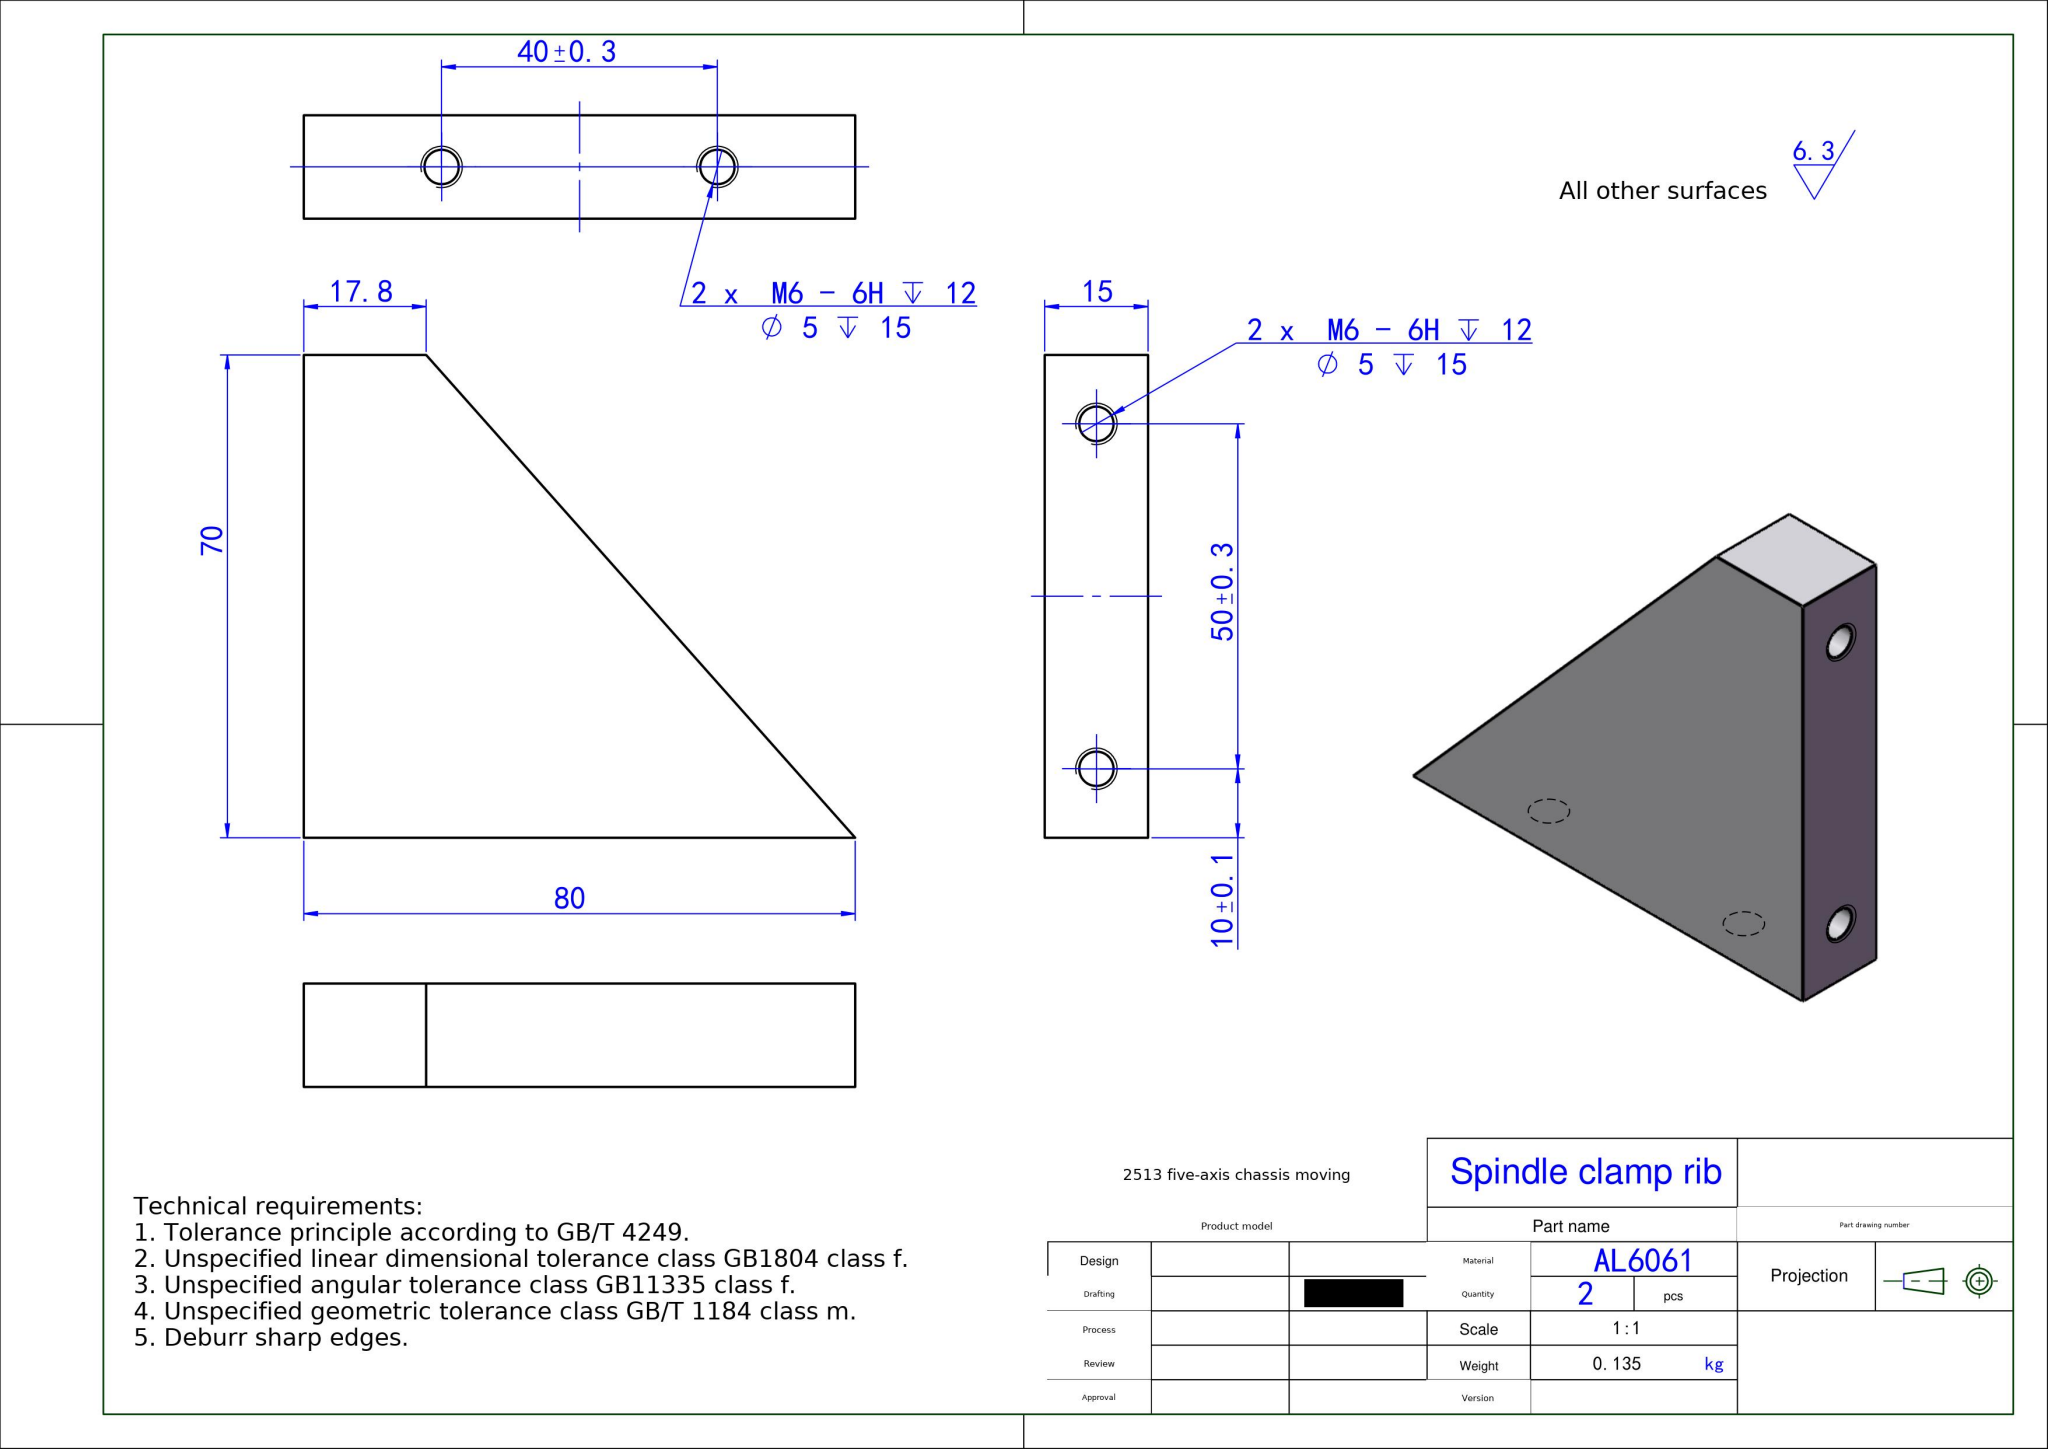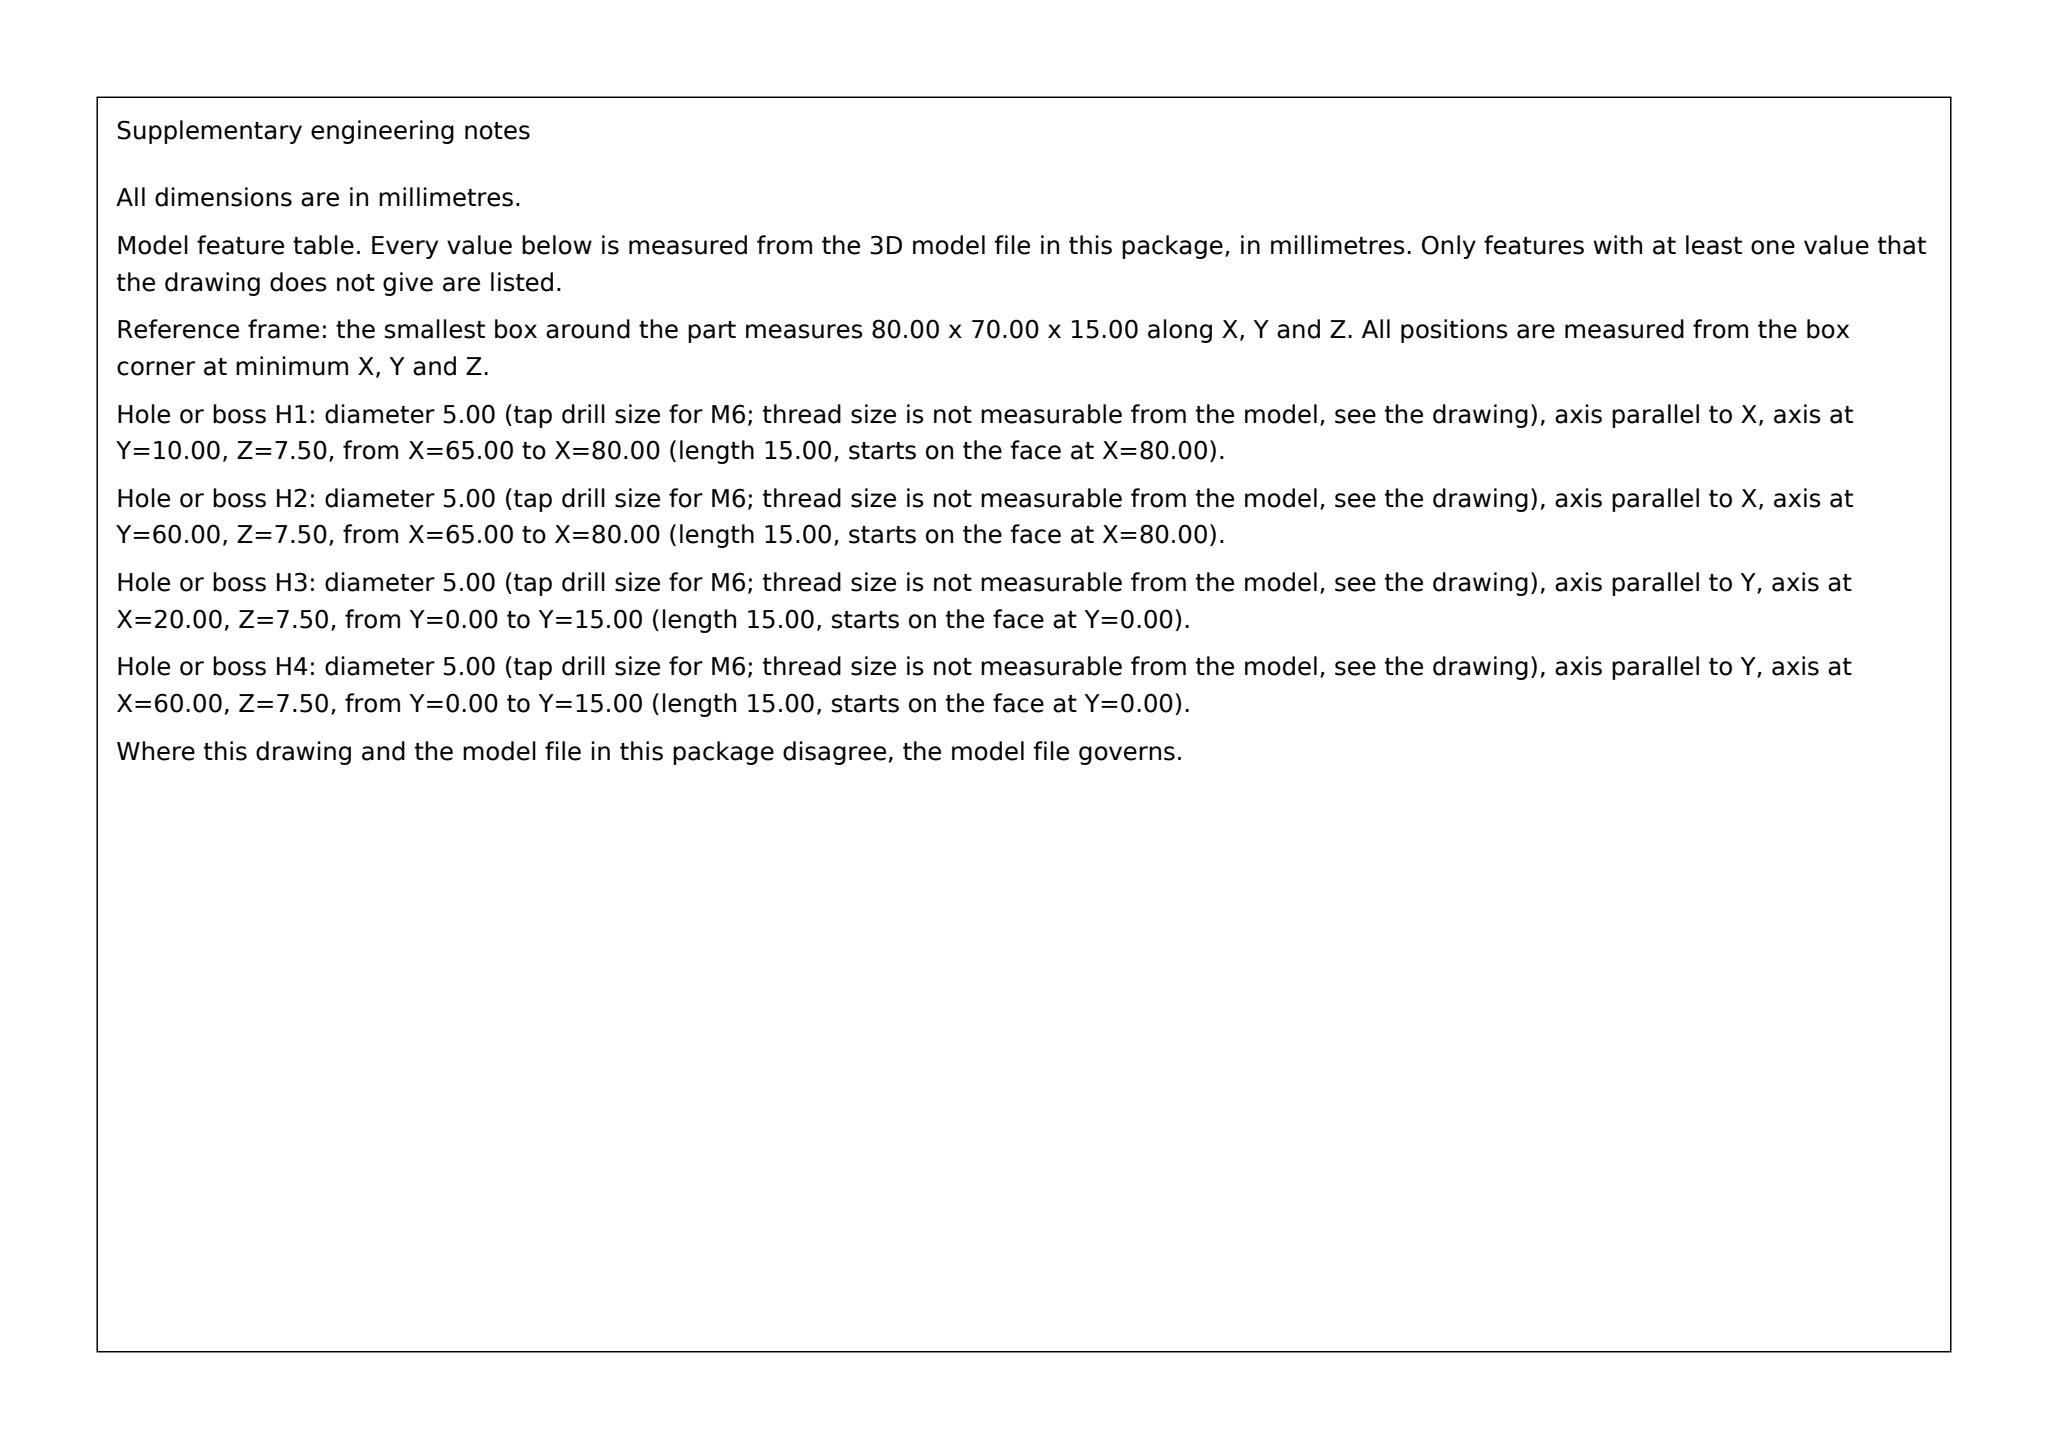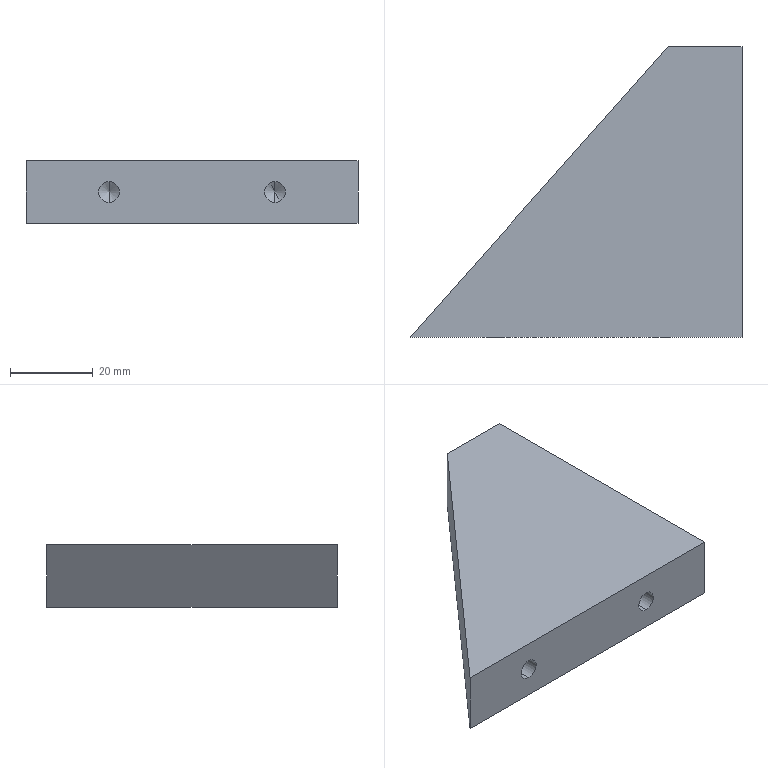Part | SolidWorks | mm | material AL6061 | 1 solid | 22 faces | box 80 x 70 x 15 mm | volume 50116 mm3 | cylinder 8 | cone 8 | plane 6 | commonest cylinder face diameters 5 x8
build123d program:
from build123d import *

# Parameters (mm, degrees)
BOSS_EXTRUDE1_DEPTH   = 15
CUT_EXTRUDE1_DEPTH    = 15
M6_TAPPED_HOLE1_D     = 5
M6_TAPPED_HOLE1_DEPTH = 15
M6_TAPPED_HOLE1_TIP   = 1.502
M6_TAPPED_HOLE2_D     = 5
M6_TAPPED_HOLE2_DEPTH = 15
M6_TAPPED_HOLE2_TIP   = 1.502


with BuildPart() as part:
    # Sketch1 → Boss-Extrude1 (new body)
    with BuildSketch(Plane.XY):
        Polygon((-23, -46), (-103, -136), (-23, -136), align=None)
    extrude(amount=-BOSS_EXTRUDE1_DEPTH)

    # Sketch2 → Cut-Extrude1 (cut)
    with BuildSketch(Plane.XY):
        Polygon((-40.778, -66), (-23, -66), (-23, -46), align=None)
    extrude(amount=-CUT_EXTRUDE1_DEPTH, mode=Mode.SUBTRACT)

    # M6 Tapped Hole1
    with Locations(Plane(origin=(-23, 0, 0), x_dir=(0, 0, -1), z_dir=(1, 0, 0))):
        with Locations((7.5, -76), (7.5, -126)):
            Hole(M6_TAPPED_HOLE1_D / 2, depth=M6_TAPPED_HOLE1_DEPTH)
            with Locations((0, 0, -(M6_TAPPED_HOLE1_DEPTH + M6_TAPPED_HOLE1_TIP / 2))):  # 118° drill point
                Cone(0, M6_TAPPED_HOLE1_D / 2, M6_TAPPED_HOLE1_TIP, mode=Mode.SUBTRACT)

    # M6 Tapped Hole2
    with Locations(Plane(origin=(0, -136, 0), x_dir=(-1, 0, 0), z_dir=(0, -1, 0))):
        with Locations((43, 7.5), (83, 7.5)):
            Hole(M6_TAPPED_HOLE2_D / 2, depth=M6_TAPPED_HOLE2_DEPTH)
            with Locations((0, 0, -(M6_TAPPED_HOLE2_DEPTH + M6_TAPPED_HOLE2_TIP / 2))):  # 118° drill point
                Cone(0, M6_TAPPED_HOLE2_D / 2, M6_TAPPED_HOLE2_TIP, mode=Mode.SUBTRACT)


solid = part.part
STEP:
#1=CARTESIAN_POINT('',(-43.,-121.,-5.));
#2=VERTEX_POINT('',#1);
#3=CARTESIAN_POINT('',(-43.,-121.,-10.));
#4=VERTEX_POINT('',#3);
#5=CARTESIAN_POINT('',(-43.,-121.,-7.5));
#6=DIRECTION('',(0.,-1.,0.));
#7=DIRECTION('',(0.,0.,-1.));
#8=AXIS2_PLACEMENT_3D('',#5,#6,#7);
#9=CIRCLE('',#8,2.5);
#10=EDGE_CURVE('',#2,#4,#9,.T.);
#11=ORIENTED_EDGE('',*,*,#10,.F.);
#12=CARTESIAN_POINT('',(-43.,-136.,-5.));
#13=VERTEX_POINT('',#12);
#14=CARTESIAN_POINT('',(-43.,-136.,-5.));
#15=DIRECTION('',(0.,-1.,0.));
#16=VECTOR('',#15,1000.);
#17=LINE('',#14,#16);
#18=EDGE_CURVE('',#2,#13,#17,.T.);
#19=ORIENTED_EDGE('',*,*,#18,.T.);
#20=CARTESIAN_POINT('',(-43.,-136.,-10.));
#21=VERTEX_POINT('',#20);
#22=CARTESIAN_POINT('',(-43.,-136.,-7.5));
#23=DIRECTION('',(0.,-1.,0.));
#24=DIRECTION('',(0.,0.,-1.));
#25=AXIS2_PLACEMENT_3D('',#22,#23,#24);
#26=CIRCLE('',#25,2.5);
#27=EDGE_CURVE('',#13,#21,#26,.T.);
#28=ORIENTED_EDGE('',*,*,#27,.T.);
#29=CARTESIAN_POINT('',(-43.,-136.,-10.));
#30=DIRECTION('',(0.,-1.,0.));
#31=VECTOR('',#30,1000.);
#32=LINE('',#29,#31);
#33=EDGE_CURVE('',#4,#21,#32,.T.);
#34=ORIENTED_EDGE('',*,*,#33,.F.);
#35=EDGE_LOOP('',(#11,#19,#28,#34));
#36=FACE_OUTER_BOUND('',#35,.T.);
#37=CARTESIAN_POINT('',(-43.,-136.,-7.5));
#38=DIRECTION('',(0.,-1.,0.));
#39=DIRECTION('',(0.,0.,-1.));
#40=AXIS2_PLACEMENT_3D('',#37,#38,#39);
#41=CYLINDRICAL_SURFACE('',#40,2.5);
#42=ADVANCED_FACE('',(#36),#41,.F.);
#43=CARTESIAN_POINT('',(-43.,-119.498,-7.5));
#44=VERTEX_POINT('',#43);
#45=CARTESIAN_POINT('',(-43.,-121.,-10.));
#46=DIRECTION('',(0.,-0.515,-0.8572));
#47=VECTOR('',#46,1000.);
#48=LINE('',#45,#47);
#49=EDGE_CURVE('',#44,#4,#48,.T.);
#50=ORIENTED_EDGE('',*,*,#49,.F.);
#51=CARTESIAN_POINT('',(-43.,-121.,-5.));
#52=DIRECTION('',(0.,-0.515,0.8572));
#53=VECTOR('',#52,1000.);
#54=LINE('',#51,#53);
#55=EDGE_CURVE('',#44,#2,#54,.T.);
#56=ORIENTED_EDGE('',*,*,#55,.T.);
#57=ORIENTED_EDGE('',*,*,#10,.T.);
#58=EDGE_LOOP('',(#50,#56,#57));
#59=FACE_OUTER_BOUND('',#58,.T.);
#60=CARTESIAN_POINT('',(-43.,-121.,-7.5));
#61=DIRECTION('',(0.,-1.,0.));
#62=DIRECTION('',(0.,0.,-1.));
#63=AXIS2_PLACEMENT_3D('',#60,#61,#62);
#64=CONICAL_SURFACE('',#63,2.5,1.03);
#65=ADVANCED_FACE('',(#59),#64,.F.);
#66=CARTESIAN_POINT('',(-83.,-121.,-5.));
#67=VERTEX_POINT('',#66);
#68=CARTESIAN_POINT('',(-83.,-121.,-10.));
#69=VERTEX_POINT('',#68);
#70=CARTESIAN_POINT('',(-83.,-121.,-7.5));
#71=DIRECTION('',(0.,-1.,0.));
#72=DIRECTION('',(0.,0.,-1.));
#73=AXIS2_PLACEMENT_3D('',#70,#71,#72);
#74=CIRCLE('',#73,2.5);
#75=EDGE_CURVE('',#67,#69,#74,.T.);
#76=ORIENTED_EDGE('',*,*,#75,.F.);
#77=CARTESIAN_POINT('',(-83.,-136.,-5.));
#78=VERTEX_POINT('',#77);
#79=CARTESIAN_POINT('',(-83.,-136.,-5.));
#80=DIRECTION('',(0.,-1.,0.));
#81=VECTOR('',#80,1000.);
#82=LINE('',#79,#81);
#83=EDGE_CURVE('',#67,#78,#82,.T.);
#84=ORIENTED_EDGE('',*,*,#83,.T.);
#85=CARTESIAN_POINT('',(-83.,-136.,-10.));
#86=VERTEX_POINT('',#85);
#87=CARTESIAN_POINT('',(-83.,-136.,-7.5));
#88=DIRECTION('',(0.,-1.,0.));
#89=DIRECTION('',(0.,0.,-1.));
#90=AXIS2_PLACEMENT_3D('',#87,#88,#89);
#91=CIRCLE('',#90,2.5);
#92=EDGE_CURVE('',#78,#86,#91,.T.);
#93=ORIENTED_EDGE('',*,*,#92,.T.);
#94=CARTESIAN_POINT('',(-83.,-136.,-10.));
#95=DIRECTION('',(0.,-1.,0.));
#96=VECTOR('',#95,1000.);
#97=LINE('',#94,#96);
#98=EDGE_CURVE('',#69,#86,#97,.T.);
#99=ORIENTED_EDGE('',*,*,#98,.F.);
#100=EDGE_LOOP('',(#76,#84,#93,#99));
#101=FACE_OUTER_BOUND('',#100,.T.);
#102=CARTESIAN_POINT('',(-83.,-136.,-7.5));
#103=DIRECTION('',(0.,-1.,0.));
#104=DIRECTION('',(0.,0.,-1.));
#105=AXIS2_PLACEMENT_3D('',#102,#103,#104);
#106=CYLINDRICAL_SURFACE('',#105,2.5);
#107=ADVANCED_FACE('',(#101),#106,.F.);
#108=CARTESIAN_POINT('',(-83.,-119.498,-7.5));
#109=VERTEX_POINT('',#108);
#110=CARTESIAN_POINT('',(-83.,-121.,-10.));
#111=DIRECTION('',(0.,-0.515,-0.8572));
#112=VECTOR('',#111,1000.);
#113=LINE('',#110,#112);
#114=EDGE_CURVE('',#109,#69,#113,.T.);
#115=ORIENTED_EDGE('',*,*,#114,.F.);
#116=CARTESIAN_POINT('',(-83.,-121.,-5.));
#117=DIRECTION('',(0.,-0.515,0.8572));
#118=VECTOR('',#117,1000.);
#119=LINE('',#116,#118);
#120=EDGE_CURVE('',#109,#67,#119,.T.);
#121=ORIENTED_EDGE('',*,*,#120,.T.);
#122=ORIENTED_EDGE('',*,*,#75,.T.);
#123=EDGE_LOOP('',(#115,#121,#122));
#124=FACE_OUTER_BOUND('',#123,.T.);
#125=CARTESIAN_POINT('',(-83.,-121.,-7.5));
#126=DIRECTION('',(0.,-1.,0.));
#127=DIRECTION('',(0.,0.,-1.));
#128=AXIS2_PLACEMENT_3D('',#125,#126,#127);
#129=CONICAL_SURFACE('',#128,2.5,1.03);
#130=ADVANCED_FACE('',(#124),#129,.F.);
#131=CARTESIAN_POINT('',(-38.,-76.,-5.));
#132=VERTEX_POINT('',#131);
#133=CARTESIAN_POINT('',(-38.,-76.,-10.));
#134=VERTEX_POINT('',#133);
#135=CARTESIAN_POINT('',(-38.,-76.,-7.5));
#136=DIRECTION('',(1.,0.,0.));
#137=DIRECTION('',(0.,0.,-1.));
#138=AXIS2_PLACEMENT_3D('',#135,#136,#137);
#139=CIRCLE('',#138,2.5);
#140=EDGE_CURVE('',#132,#134,#139,.T.);
#141=ORIENTED_EDGE('',*,*,#140,.F.);
#142=CARTESIAN_POINT('',(-23.,-76.,-5.));
#143=VERTEX_POINT('',#142);
#144=CARTESIAN_POINT('',(-23.,-76.,-5.));
#145=DIRECTION('',(1.,0.,0.));
#146=VECTOR('',#145,1000.);
#147=LINE('',#144,#146);
#148=EDGE_CURVE('',#132,#143,#147,.T.);
#149=ORIENTED_EDGE('',*,*,#148,.T.);
#150=CARTESIAN_POINT('',(-23.,-76.,-10.));
#151=VERTEX_POINT('',#150);
#152=CARTESIAN_POINT('',(-23.,-76.,-7.5));
#153=DIRECTION('',(1.,0.,0.));
#154=DIRECTION('',(0.,0.,-1.));
#155=AXIS2_PLACEMENT_3D('',#152,#153,#154);
#156=CIRCLE('',#155,2.5);
#157=EDGE_CURVE('',#143,#151,#156,.T.);
#158=ORIENTED_EDGE('',*,*,#157,.T.);
#159=CARTESIAN_POINT('',(-23.,-76.,-10.));
#160=DIRECTION('',(1.,0.,0.));
#161=VECTOR('',#160,1000.);
#162=LINE('',#159,#161);
#163=EDGE_CURVE('',#134,#151,#162,.T.);
#164=ORIENTED_EDGE('',*,*,#163,.F.);
#165=EDGE_LOOP('',(#141,#149,#158,#164));
#166=FACE_OUTER_BOUND('',#165,.T.);
#167=CARTESIAN_POINT('',(-23.,-76.,-7.5));
#168=DIRECTION('',(1.,0.,0.));
#169=DIRECTION('',(0.,0.,-1.));
#170=AXIS2_PLACEMENT_3D('',#167,#168,#169);
#171=CYLINDRICAL_SURFACE('',#170,2.5);
#172=ADVANCED_FACE('',(#166),#171,.F.);
#173=CARTESIAN_POINT('',(-39.502,-76.,-7.5));
#174=VERTEX_POINT('',#173);
#175=CARTESIAN_POINT('',(-38.,-76.,-10.));
#176=DIRECTION('',(0.515,0.,-0.8572));
#177=VECTOR('',#176,1000.);
#178=LINE('',#175,#177);
#179=EDGE_CURVE('',#174,#134,#178,.T.);
#180=ORIENTED_EDGE('',*,*,#179,.F.);
#181=CARTESIAN_POINT('',(-38.,-76.,-5.));
#182=DIRECTION('',(0.515,0.,0.8572));
#183=VECTOR('',#182,1000.);
#184=LINE('',#181,#183);
#185=EDGE_CURVE('',#174,#132,#184,.T.);
#186=ORIENTED_EDGE('',*,*,#185,.T.);
#187=ORIENTED_EDGE('',*,*,#140,.T.);
#188=EDGE_LOOP('',(#180,#186,#187));
#189=FACE_OUTER_BOUND('',#188,.T.);
#190=CARTESIAN_POINT('',(-38.,-76.,-7.5));
#191=DIRECTION('',(1.,0.,0.));
#192=DIRECTION('',(0.,0.,-1.));
#193=AXIS2_PLACEMENT_3D('',#190,#191,#192);
#194=CONICAL_SURFACE('',#193,2.5,1.03);
#195=ADVANCED_FACE('',(#189),#194,.F.);
#196=CARTESIAN_POINT('',(-38.,-126.,-5.));
#197=VERTEX_POINT('',#196);
#198=CARTESIAN_POINT('',(-38.,-126.,-10.));
#199=VERTEX_POINT('',#198);
#200=CARTESIAN_POINT('',(-38.,-126.,-7.5));
#201=DIRECTION('',(1.,0.,0.));
#202=DIRECTION('',(0.,0.,-1.));
#203=AXIS2_PLACEMENT_3D('',#200,#201,#202);
#204=CIRCLE('',#203,2.5);
#205=EDGE_CURVE('',#197,#199,#204,.T.);
#206=ORIENTED_EDGE('',*,*,#205,.F.);
#207=CARTESIAN_POINT('',(-23.,-126.,-5.));
#208=VERTEX_POINT('',#207);
#209=CARTESIAN_POINT('',(-23.,-126.,-5.));
#210=DIRECTION('',(1.,0.,0.));
#211=VECTOR('',#210,1000.);
#212=LINE('',#209,#211);
#213=EDGE_CURVE('',#197,#208,#212,.T.);
#214=ORIENTED_EDGE('',*,*,#213,.T.);
#215=CARTESIAN_POINT('',(-23.,-126.,-10.));
#216=VERTEX_POINT('',#215);
#217=CARTESIAN_POINT('',(-23.,-126.,-7.5));
#218=DIRECTION('',(1.,0.,0.));
#219=DIRECTION('',(0.,0.,-1.));
#220=AXIS2_PLACEMENT_3D('',#217,#218,#219);
#221=CIRCLE('',#220,2.5);
#222=EDGE_CURVE('',#208,#216,#221,.T.);
#223=ORIENTED_EDGE('',*,*,#222,.T.);
#224=CARTESIAN_POINT('',(-23.,-126.,-10.));
#225=DIRECTION('',(1.,0.,0.));
#226=VECTOR('',#225,1000.);
#227=LINE('',#224,#226);
#228=EDGE_CURVE('',#199,#216,#227,.T.);
#229=ORIENTED_EDGE('',*,*,#228,.F.);
#230=EDGE_LOOP('',(#206,#214,#223,#229));
#231=FACE_OUTER_BOUND('',#230,.T.);
#232=CARTESIAN_POINT('',(-23.,-126.,-7.5));
#233=DIRECTION('',(1.,0.,0.));
#234=DIRECTION('',(0.,0.,-1.));
#235=AXIS2_PLACEMENT_3D('',#232,#233,#234);
#236=CYLINDRICAL_SURFACE('',#235,2.5);
#237=ADVANCED_FACE('',(#231),#236,.F.);
#238=CARTESIAN_POINT('',(-39.502,-126.,-7.5));
#239=VERTEX_POINT('',#238);
#240=CARTESIAN_POINT('',(-38.,-126.,-10.));
#241=DIRECTION('',(0.515,0.,-0.8572));
#242=VECTOR('',#241,1000.);
#243=LINE('',#240,#242);
#244=EDGE_CURVE('',#239,#199,#243,.T.);
#245=ORIENTED_EDGE('',*,*,#244,.F.);
#246=CARTESIAN_POINT('',(-38.,-126.,-5.));
#247=DIRECTION('',(0.515,0.,0.8572));
#248=VECTOR('',#247,1000.);
#249=LINE('',#246,#248);
#250=EDGE_CURVE('',#239,#197,#249,.T.);
#251=ORIENTED_EDGE('',*,*,#250,.T.);
#252=ORIENTED_EDGE('',*,*,#205,.T.);
#253=EDGE_LOOP('',(#245,#251,#252));
#254=FACE_OUTER_BOUND('',#253,.T.);
#255=CARTESIAN_POINT('',(-38.,-126.,-7.5));
#256=DIRECTION('',(1.,0.,0.));
#257=DIRECTION('',(0.,0.,-1.));
#258=AXIS2_PLACEMENT_3D('',#255,#256,#257);
#259=CONICAL_SURFACE('',#258,2.5,1.03);
#260=ADVANCED_FACE('',(#254),#259,.F.);
#261=CARTESIAN_POINT('',(-23.,-76.,-7.5));
#262=DIRECTION('',(1.,0.,0.));
#263=DIRECTION('',(0.,0.,-1.));
#264=AXIS2_PLACEMENT_3D('',#261,#262,#263);
#265=CIRCLE('',#264,2.5);
#266=EDGE_CURVE('',#151,#143,#265,.T.);
#267=ORIENTED_EDGE('',*,*,#266,.F.);
#268=ORIENTED_EDGE('',*,*,#157,.F.);
#269=EDGE_LOOP('',(#267,#268));
#270=FACE_BOUND('',#269,.T.);
#271=CARTESIAN_POINT('',(-23.,-126.,-7.5));
#272=DIRECTION('',(1.,0.,0.));
#273=DIRECTION('',(0.,0.,-1.));
#274=AXIS2_PLACEMENT_3D('',#271,#272,#273);
#275=CIRCLE('',#274,2.5);
#276=EDGE_CURVE('',#216,#208,#275,.T.);
#277=ORIENTED_EDGE('',*,*,#276,.F.);
#278=ORIENTED_EDGE('',*,*,#222,.F.);
#279=EDGE_LOOP('',(#277,#278));
#280=FACE_BOUND('',#279,.T.);
#281=CARTESIAN_POINT('',(-23.,-66.,-15.));
#282=VERTEX_POINT('',#281);
#283=CARTESIAN_POINT('',(-23.,-66.,0.));
#284=VERTEX_POINT('',#283);
#285=CARTESIAN_POINT('',(-23.,-66.,-41.759));
#286=DIRECTION('',(0.,0.,1.));
#287=VECTOR('',#286,1000.);
#288=LINE('',#285,#287);
#289=EDGE_CURVE('',#282,#284,#288,.T.);
#290=ORIENTED_EDGE('',*,*,#289,.T.);
#291=CARTESIAN_POINT('',(-23.,-136.,0.));
#292=VERTEX_POINT('',#291);
#293=CARTESIAN_POINT('',(-23.,-136.,0.));
#294=DIRECTION('',(0.,1.,0.));
#295=VECTOR('',#294,1000.);
#296=LINE('',#293,#295);
#297=EDGE_CURVE('',#292,#284,#296,.T.);
#298=ORIENTED_EDGE('',*,*,#297,.F.);
#299=CARTESIAN_POINT('',(-23.,-136.,-15.));
#300=VERTEX_POINT('',#299);
#301=CARTESIAN_POINT('',(-23.,-136.,-15.));
#302=DIRECTION('',(0.,0.,1.));
#303=VECTOR('',#302,1000.);
#304=LINE('',#301,#303);
#305=EDGE_CURVE('',#300,#292,#304,.T.);
#306=ORIENTED_EDGE('',*,*,#305,.F.);
#307=CARTESIAN_POINT('',(-23.,-136.,-15.));
#308=DIRECTION('',(0.,1.,0.));
#309=VECTOR('',#308,1000.);
#310=LINE('',#307,#309);
#311=EDGE_CURVE('',#300,#282,#310,.T.);
#312=ORIENTED_EDGE('',*,*,#311,.T.);
#313=EDGE_LOOP('',(#290,#298,#306,#312));
#314=FACE_OUTER_BOUND('',#313,.T.);
#315=CARTESIAN_POINT('',(-23.,-136.,-15.));
#316=DIRECTION('',(1.,-0.,0.));
#317=DIRECTION('',(0.,1.,0.));
#318=AXIS2_PLACEMENT_3D('',#315,#316,#317);
#319=PLANE('',#318);
#320=ADVANCED_FACE('',(#270,#280,#314),#319,.T.);
#321=CARTESIAN_POINT('',(-43.,-136.,-7.5));
#322=DIRECTION('',(0.,-1.,0.));
#323=DIRECTION('',(0.,0.,-1.));
#324=AXIS2_PLACEMENT_3D('',#321,#322,#323);
#325=CIRCLE('',#324,2.5);
#326=EDGE_CURVE('',#21,#13,#325,.T.);
#327=ORIENTED_EDGE('',*,*,#326,.F.);
#328=ORIENTED_EDGE('',*,*,#27,.F.);
#329=EDGE_LOOP('',(#327,#328));
#330=FACE_BOUND('',#329,.T.);
#331=CARTESIAN_POINT('',(-83.,-136.,-7.5));
#332=DIRECTION('',(0.,-1.,0.));
#333=DIRECTION('',(0.,0.,-1.));
#334=AXIS2_PLACEMENT_3D('',#331,#332,#333);
#335=CIRCLE('',#334,2.5);
#336=EDGE_CURVE('',#86,#78,#335,.T.);
#337=ORIENTED_EDGE('',*,*,#336,.F.);
#338=ORIENTED_EDGE('',*,*,#92,.F.);
#339=EDGE_LOOP('',(#337,#338));
#340=FACE_BOUND('',#339,.T.);
#341=CARTESIAN_POINT('',(-103.,-136.,0.));
#342=VERTEX_POINT('',#341);
#343=CARTESIAN_POINT('',(-103.,-136.,0.));
#344=DIRECTION('',(1.,0.,0.));
#345=VECTOR('',#344,1000.);
#346=LINE('',#343,#345);
#347=EDGE_CURVE('',#342,#292,#346,.T.);
#348=ORIENTED_EDGE('',*,*,#347,.F.);
#349=CARTESIAN_POINT('',(-103.,-136.,-15.));
#350=VERTEX_POINT('',#349);
#351=CARTESIAN_POINT('',(-103.,-136.,-15.));
#352=DIRECTION('',(0.,0.,1.));
#353=VECTOR('',#352,1000.);
#354=LINE('',#351,#353);
#355=EDGE_CURVE('',#350,#342,#354,.T.);
#356=ORIENTED_EDGE('',*,*,#355,.F.);
#357=CARTESIAN_POINT('',(-103.,-136.,-15.));
#358=DIRECTION('',(1.,0.,0.));
#359=VECTOR('',#358,1000.);
#360=LINE('',#357,#359);
#361=EDGE_CURVE('',#350,#300,#360,.T.);
#362=ORIENTED_EDGE('',*,*,#361,.T.);
#363=ORIENTED_EDGE('',*,*,#305,.T.);
#364=EDGE_LOOP('',(#348,#356,#362,#363));
#365=FACE_OUTER_BOUND('',#364,.T.);
#366=CARTESIAN_POINT('',(-103.,-136.,-15.));
#367=DIRECTION('',(0.,-1.,0.));
#368=DIRECTION('',(0.,0.,-1.));
#369=AXIS2_PLACEMENT_3D('',#366,#367,#368);
#370=PLANE('',#369);
#371=ADVANCED_FACE('',(#330,#340,#365),#370,.T.);
#372=CARTESIAN_POINT('',(-40.778,-66.,-15.));
#373=VERTEX_POINT('',#372);
#374=CARTESIAN_POINT('',(-40.778,-66.,0.));
#375=VERTEX_POINT('',#374);
#376=CARTESIAN_POINT('',(-40.778,-66.,-41.759));
#377=DIRECTION('',(0.,0.,1.));
#378=VECTOR('',#377,1000.);
#379=LINE('',#376,#378);
#380=EDGE_CURVE('',#373,#375,#379,.T.);
#381=ORIENTED_EDGE('',*,*,#380,.F.);
#382=CARTESIAN_POINT('',(-23.,-46.,-15.));
#383=DIRECTION('',(-0.6644,-0.7474,0.));
#384=VECTOR('',#383,1000.);
#385=LINE('',#382,#384);
#386=EDGE_CURVE('',#373,#350,#385,.T.);
#387=ORIENTED_EDGE('',*,*,#386,.T.);
#388=ORIENTED_EDGE('',*,*,#355,.T.);
#389=CARTESIAN_POINT('',(-23.,-46.,0.));
#390=DIRECTION('',(-0.6644,-0.7474,0.));
#391=VECTOR('',#390,1000.);
#392=LINE('',#389,#391);
#393=EDGE_CURVE('',#375,#342,#392,.T.);
#394=ORIENTED_EDGE('',*,*,#393,.F.);
#395=EDGE_LOOP('',(#381,#387,#388,#394));
#396=FACE_OUTER_BOUND('',#395,.T.);
#397=CARTESIAN_POINT('',(-23.,-46.,-15.));
#398=DIRECTION('',(-0.7474,0.6644,0.));
#399=DIRECTION('',(-0.6644,-0.7474,0.));
#400=AXIS2_PLACEMENT_3D('',#397,#398,#399);
#401=PLANE('',#400);
#402=ADVANCED_FACE('',(#396),#401,.T.);
#403=CARTESIAN_POINT('',(-40.778,-66.,-15.));
#404=DIRECTION('',(1.,0.,0.));
#405=VECTOR('',#404,1000.);
#406=LINE('',#403,#405);
#407=EDGE_CURVE('',#373,#282,#406,.T.);
#408=ORIENTED_EDGE('',*,*,#407,.T.);
#409=ORIENTED_EDGE('',*,*,#311,.F.);
#410=ORIENTED_EDGE('',*,*,#361,.F.);
#411=ORIENTED_EDGE('',*,*,#386,.F.);
#412=EDGE_LOOP('',(#408,#409,#410,#411));
#413=FACE_OUTER_BOUND('',#412,.T.);
#414=CARTESIAN_POINT('',(0.,0.,-15.));
#415=DIRECTION('',(0.,0.,-1.));
#416=DIRECTION('',(-1.,0.,0.));
#417=AXIS2_PLACEMENT_3D('',#414,#415,#416);
#418=PLANE('',#417);
#419=ADVANCED_FACE('',(#413),#418,.T.);
#420=ORIENTED_EDGE('',*,*,#297,.T.);
#421=CARTESIAN_POINT('',(-40.778,-66.,0.));
#422=DIRECTION('',(1.,0.,0.));
#423=VECTOR('',#422,1000.);
#424=LINE('',#421,#423);
#425=EDGE_CURVE('',#375,#284,#424,.T.);
#426=ORIENTED_EDGE('',*,*,#425,.F.);
#427=ORIENTED_EDGE('',*,*,#393,.T.);
#428=ORIENTED_EDGE('',*,*,#347,.T.);
#429=EDGE_LOOP('',(#420,#426,#427,#428));
#430=FACE_OUTER_BOUND('',#429,.T.);
#431=CARTESIAN_POINT('',(0.,0.,0.));
#432=DIRECTION('',(0.,0.,-1.));
#433=DIRECTION('',(-1.,0.,0.));
#434=AXIS2_PLACEMENT_3D('',#431,#432,#433);
#435=PLANE('',#434);
#436=ADVANCED_FACE('',(#430),#435,.F.);
#437=ORIENTED_EDGE('',*,*,#380,.T.);
#438=ORIENTED_EDGE('',*,*,#425,.T.);
#439=ORIENTED_EDGE('',*,*,#289,.F.);
#440=ORIENTED_EDGE('',*,*,#407,.F.);
#441=EDGE_LOOP('',(#437,#438,#439,#440));
#442=FACE_OUTER_BOUND('',#441,.T.);
#443=CARTESIAN_POINT('',(-40.778,-66.,-41.759));
#444=DIRECTION('',(0.,-1.,0.));
#445=DIRECTION('',(0.,0.,-1.));
#446=AXIS2_PLACEMENT_3D('',#443,#444,#445);
#447=PLANE('',#446);
#448=ADVANCED_FACE('',(#442),#447,.F.);
#449=ORIENTED_EDGE('',*,*,#250,.F.);
#450=ORIENTED_EDGE('',*,*,#244,.T.);
#451=CARTESIAN_POINT('',(-38.,-126.,-7.5));
#452=DIRECTION('',(1.,0.,0.));
#453=DIRECTION('',(0.,0.,-1.));
#454=AXIS2_PLACEMENT_3D('',#451,#452,#453);
#455=CIRCLE('',#454,2.5);
#456=EDGE_CURVE('',#199,#197,#455,.T.);
#457=ORIENTED_EDGE('',*,*,#456,.T.);
#458=EDGE_LOOP('',(#449,#450,#457));
#459=FACE_OUTER_BOUND('',#458,.T.);
#460=CARTESIAN_POINT('',(-38.,-126.,-7.5));
#461=DIRECTION('',(1.,0.,0.));
#462=DIRECTION('',(0.,0.,-1.));
#463=AXIS2_PLACEMENT_3D('',#460,#461,#462);
#464=CONICAL_SURFACE('',#463,2.5,1.03);
#465=ADVANCED_FACE('',(#459),#464,.F.);
#466=ORIENTED_EDGE('',*,*,#213,.F.);
#467=ORIENTED_EDGE('',*,*,#456,.F.);
#468=ORIENTED_EDGE('',*,*,#228,.T.);
#469=ORIENTED_EDGE('',*,*,#276,.T.);
#470=EDGE_LOOP('',(#466,#467,#468,#469));
#471=FACE_OUTER_BOUND('',#470,.T.);
#472=CARTESIAN_POINT('',(-23.,-126.,-7.5));
#473=DIRECTION('',(1.,0.,0.));
#474=DIRECTION('',(0.,0.,-1.));
#475=AXIS2_PLACEMENT_3D('',#472,#473,#474);
#476=CYLINDRICAL_SURFACE('',#475,2.5);
#477=ADVANCED_FACE('',(#471),#476,.F.);
#478=ORIENTED_EDGE('',*,*,#185,.F.);
#479=ORIENTED_EDGE('',*,*,#179,.T.);
#480=CARTESIAN_POINT('',(-38.,-76.,-7.5));
#481=DIRECTION('',(1.,0.,0.));
#482=DIRECTION('',(0.,0.,-1.));
#483=AXIS2_PLACEMENT_3D('',#480,#481,#482);
#484=CIRCLE('',#483,2.5);
#485=EDGE_CURVE('',#134,#132,#484,.T.);
#486=ORIENTED_EDGE('',*,*,#485,.T.);
#487=EDGE_LOOP('',(#478,#479,#486));
#488=FACE_OUTER_BOUND('',#487,.T.);
#489=CARTESIAN_POINT('',(-38.,-76.,-7.5));
#490=DIRECTION('',(1.,0.,0.));
#491=DIRECTION('',(0.,0.,-1.));
#492=AXIS2_PLACEMENT_3D('',#489,#490,#491);
#493=CONICAL_SURFACE('',#492,2.5,1.03);
#494=ADVANCED_FACE('',(#488),#493,.F.);
#495=ORIENTED_EDGE('',*,*,#148,.F.);
#496=ORIENTED_EDGE('',*,*,#485,.F.);
#497=ORIENTED_EDGE('',*,*,#163,.T.);
#498=ORIENTED_EDGE('',*,*,#266,.T.);
#499=EDGE_LOOP('',(#495,#496,#497,#498));
#500=FACE_OUTER_BOUND('',#499,.T.);
#501=CARTESIAN_POINT('',(-23.,-76.,-7.5));
#502=DIRECTION('',(1.,0.,0.));
#503=DIRECTION('',(0.,0.,-1.));
#504=AXIS2_PLACEMENT_3D('',#501,#502,#503);
#505=CYLINDRICAL_SURFACE('',#504,2.5);
#506=ADVANCED_FACE('',(#500),#505,.F.);
#507=ORIENTED_EDGE('',*,*,#120,.F.);
#508=ORIENTED_EDGE('',*,*,#114,.T.);
#509=CARTESIAN_POINT('',(-83.,-121.,-7.5));
#510=DIRECTION('',(0.,-1.,0.));
#511=DIRECTION('',(0.,0.,-1.));
#512=AXIS2_PLACEMENT_3D('',#509,#510,#511);
#513=CIRCLE('',#512,2.5);
#514=EDGE_CURVE('',#69,#67,#513,.T.);
#515=ORIENTED_EDGE('',*,*,#514,.T.);
#516=EDGE_LOOP('',(#507,#508,#515));
#517=FACE_OUTER_BOUND('',#516,.T.);
#518=CARTESIAN_POINT('',(-83.,-121.,-7.5));
#519=DIRECTION('',(0.,-1.,0.));
#520=DIRECTION('',(0.,0.,-1.));
#521=AXIS2_PLACEMENT_3D('',#518,#519,#520);
#522=CONICAL_SURFACE('',#521,2.5,1.03);
#523=ADVANCED_FACE('',(#517),#522,.F.);
#524=ORIENTED_EDGE('',*,*,#83,.F.);
#525=ORIENTED_EDGE('',*,*,#514,.F.);
#526=ORIENTED_EDGE('',*,*,#98,.T.);
#527=ORIENTED_EDGE('',*,*,#336,.T.);
#528=EDGE_LOOP('',(#524,#525,#526,#527));
#529=FACE_OUTER_BOUND('',#528,.T.);
#530=CARTESIAN_POINT('',(-83.,-136.,-7.5));
#531=DIRECTION('',(0.,-1.,0.));
#532=DIRECTION('',(0.,0.,-1.));
#533=AXIS2_PLACEMENT_3D('',#530,#531,#532);
#534=CYLINDRICAL_SURFACE('',#533,2.5);
#535=ADVANCED_FACE('',(#529),#534,.F.);
#536=ORIENTED_EDGE('',*,*,#55,.F.);
#537=ORIENTED_EDGE('',*,*,#49,.T.);
#538=CARTESIAN_POINT('',(-43.,-121.,-7.5));
#539=DIRECTION('',(0.,-1.,0.));
#540=DIRECTION('',(0.,0.,-1.));
#541=AXIS2_PLACEMENT_3D('',#538,#539,#540);
#542=CIRCLE('',#541,2.5);
#543=EDGE_CURVE('',#4,#2,#542,.T.);
#544=ORIENTED_EDGE('',*,*,#543,.T.);
#545=EDGE_LOOP('',(#536,#537,#544));
#546=FACE_OUTER_BOUND('',#545,.T.);
#547=CARTESIAN_POINT('',(-43.,-121.,-7.5));
#548=DIRECTION('',(0.,-1.,0.));
#549=DIRECTION('',(0.,0.,-1.));
#550=AXIS2_PLACEMENT_3D('',#547,#548,#549);
#551=CONICAL_SURFACE('',#550,2.5,1.03);
#552=ADVANCED_FACE('',(#546),#551,.F.);
#553=ORIENTED_EDGE('',*,*,#18,.F.);
#554=ORIENTED_EDGE('',*,*,#543,.F.);
#555=ORIENTED_EDGE('',*,*,#33,.T.);
#556=ORIENTED_EDGE('',*,*,#326,.T.);
#557=EDGE_LOOP('',(#553,#554,#555,#556));
#558=FACE_OUTER_BOUND('',#557,.T.);
#559=CARTESIAN_POINT('',(-43.,-136.,-7.5));
#560=DIRECTION('',(0.,-1.,0.));
#561=DIRECTION('',(0.,0.,-1.));
#562=AXIS2_PLACEMENT_3D('',#559,#560,#561);
#563=CYLINDRICAL_SURFACE('',#562,2.5);
#564=ADVANCED_FACE('',(#558),#563,.F.);
#565=CLOSED_SHELL('',(#42,#65,#107,#130,#172,#195,#237,#260,#320,#371,#402,#419,#436,#448,#465,#477,#494,#506,#523,#535,#552,#564));
#566=MANIFOLD_SOLID_BREP('',#565);
#567=CARTESIAN_POINT('',(0.,0.,0.));
#568=DIRECTION('',(0.,0.,1.));
#569=DIRECTION('',(1.,0.,0.));
#570=AXIS2_PLACEMENT_3D('',#567,#568,#569);
#571=(LENGTH_UNIT()NAMED_UNIT(*)SI_UNIT(.MILLI.,.METRE.));
#572=UNCERTAINTY_MEASURE_WITH_UNIT(LENGTH_MEASURE(0.00001),#571,'','');
#573=(NAMED_UNIT(*)PLANE_ANGLE_UNIT()SI_UNIT($,.RADIAN.));
#574=(NAMED_UNIT(*)SI_UNIT($,.STERADIAN.)SOLID_ANGLE_UNIT());
#575=(GEOMETRIC_REPRESENTATION_CONTEXT(3)GLOBAL_UNCERTAINTY_ASSIGNED_CONTEXT((#572))GLOBAL_UNIT_ASSIGNED_CONTEXT((#571,#573,#574))REPRESENTATION_CONTEXT('',''));
#576=ADVANCED_BREP_SHAPE_REPRESENTATION('',(#566,#570),#575);